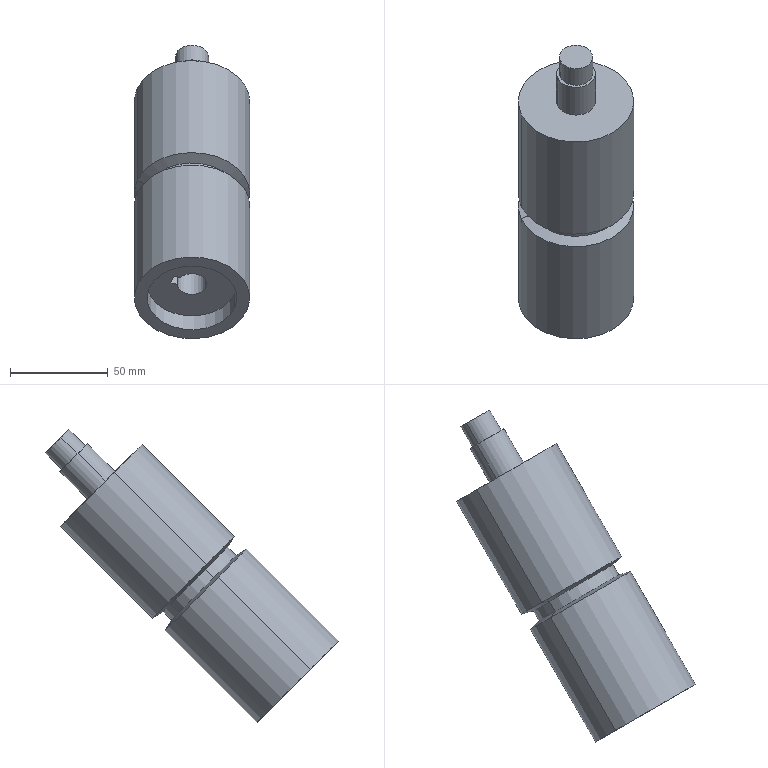Component | SolidWorks | AssemblyDriveAxis-1_DriveRoller-1 | 1 solid | 26 faces | box 59 x 149.91 x 149.91 mm | volume 368541 mm3 | cylinder 13 | plane 9 | cone 4 | commonest cylinder face diameters 59 x4 46 x2 47 x2 20 x2 17 x2 15 x1
build123d program:
from build123d import *

# Parameters (mm, degrees)
SKETCH2_W          = 5
SKETCH2_H          = 6.09
CUT_EXTRUDE1_DEPTH = 23.5


with BuildPart() as part:
    # Sketch1 → Revolve1 (revolve)
    with BuildSketch(Plane.XY, mode=Mode.PRIVATE) as revolve1_sk:
        Polygon((0, 0), (0, 8.5), (12, 8.5), (12, 10), (32, 10), (32, 29.5), (98.5, 29.5), (100, 23.5), (106, 23.5), (107.5, 29.5), (174, 29.5), (174, 23), (164, 23), (164, 7.5), (140.5, 7.5), (140.5, 0), align=None)
    revolve(revolve1_sk.sketch.rotate(Axis((0, 0, 0), (1, 0, 0)), 180), axis=Axis((0, 0, 0), (1, 0, 0)))

    # Sketch2 → Cut-Extrude1 (cut)
    with BuildSketch(Plane(origin=(164, 0, 0), x_dir=(0, 0, -1), z_dir=(1, 0, 0))):
        with Locations((0, -7.455)):
            Rectangle(SKETCH2_W, SKETCH2_H)
    extrude(amount=-CUT_EXTRUDE1_DEPTH, mode=Mode.SUBTRACT)


solid = part.part

# Placed as in the assembly
solid = solid.moved(Location((-102, 782.054, 414.962), (45, 18.175, -90)))
STEP:
#1=COLOUR_RGB('',0.7922,0.8196,0.9333);
#2=FILL_AREA_STYLE_COLOUR('',#1);
#3=FILL_AREA_STYLE('',(#2));
#4=SURFACE_STYLE_FILL_AREA(#3);
#5=SURFACE_SIDE_STYLE('',(#4));
#6=SURFACE_STYLE_USAGE(.BOTH.,#5);
#7=PRESENTATION_STYLE_ASSIGNMENT((#6));
#8=CARTESIAN_POINT('',(-3.155,26.145,11.293));
#9=VERTEX_POINT('',#8);
#10=CARTESIAN_POINT('',(-4.876,25.746,11.693));
#11=VERTEX_POINT('',#10);
#12=CARTESIAN_POINT('',(-4.016,25.946,11.493));
#13=DIRECTION('',(-0.,0.7071,0.7071));
#14=DIRECTION('',(-0.9501,-0.2206,0.2206));
#15=AXIS2_PLACEMENT_3D('',#12,#13,#14);
#16=CIRCLE('',#15,0.9055);
#17=EDGE_CURVE('',#9,#11,#16,.T.);
#18=ORIENTED_EDGE('',*,*,#17,.F.);
#19=CARTESIAN_POINT('',(-3.155,26.424,11.572));
#20=VERTEX_POINT('',#19);
#21=CARTESIAN_POINT('',(-3.155,30.989,16.137));
#22=DIRECTION('',(-0.,0.7071,0.7071));
#23=VECTOR('',#22,39.37);
#24=LINE('',#21,#23);
#25=EDGE_CURVE('',#9,#20,#24,.T.);
#26=ORIENTED_EDGE('',*,*,#25,.T.);
#27=CARTESIAN_POINT('',(-4.876,26.024,11.971));
#28=VERTEX_POINT('',#27);
#29=CARTESIAN_POINT('',(-4.016,26.224,11.772));
#30=DIRECTION('',(-0.,0.7071,0.7071));
#31=DIRECTION('',(-0.9501,-0.2206,0.2206));
#32=AXIS2_PLACEMENT_3D('',#29,#30,#31);
#33=CIRCLE('',#32,0.9055);
#34=EDGE_CURVE('',#20,#28,#33,.T.);
#35=ORIENTED_EDGE('',*,*,#34,.T.);
#36=CARTESIAN_POINT('',(-4.876,30.59,16.537));
#37=DIRECTION('',(-0.,0.7071,0.7071));
#38=VECTOR('',#37,39.37);
#39=LINE('',#36,#38);
#40=EDGE_CURVE('',#11,#28,#39,.T.);
#41=ORIENTED_EDGE('',*,*,#40,.F.);
#42=EDGE_LOOP('',(#18,#26,#35,#41));
#43=FACE_OUTER_BOUND('',#42,.T.);
#44=CARTESIAN_POINT('',(-4.016,30.79,16.337));
#45=DIRECTION('',(-0.,0.7071,0.7071));
#46=DIRECTION('',(-0.9501,-0.2206,0.2206));
#47=AXIS2_PLACEMENT_3D('',#44,#45,#46);
#48=CYLINDRICAL_SURFACE('',#47,0.9055);
#49=ADVANCED_FACE('',(#43),#48,.F.);
#50=CARTESIAN_POINT('',(-5.119,25.689,11.749));
#51=VERTEX_POINT('',#50);
#52=CARTESIAN_POINT('',(-2.912,26.202,11.237));
#53=VERTEX_POINT('',#52);
#54=CARTESIAN_POINT('',(-4.016,25.946,11.493));
#55=DIRECTION('',(-0.,0.7071,0.7071));
#56=DIRECTION('',(-0.9501,-0.2206,0.2206));
#57=AXIS2_PLACEMENT_3D('',#54,#55,#56);
#58=CIRCLE('',#57,1.161);
#59=EDGE_CURVE('',#51,#53,#58,.T.);
#60=ORIENTED_EDGE('',*,*,#59,.T.);
#61=CARTESIAN_POINT('',(-2.912,28.053,13.088));
#62=VERTEX_POINT('',#61);
#63=CARTESIAN_POINT('',(-2.912,31.046,16.081));
#64=DIRECTION('',(-0.,0.7071,0.7071));
#65=VECTOR('',#64,39.37);
#66=LINE('',#63,#65);
#67=EDGE_CURVE('',#53,#62,#66,.T.);
#68=ORIENTED_EDGE('',*,*,#67,.T.);
#69=CARTESIAN_POINT('',(-5.119,27.541,13.601));
#70=VERTEX_POINT('',#69);
#71=CARTESIAN_POINT('',(-4.016,27.797,13.344));
#72=DIRECTION('',(-0.,0.7071,0.7071));
#73=DIRECTION('',(-0.9501,-0.2206,0.2206));
#74=AXIS2_PLACEMENT_3D('',#71,#72,#73);
#75=CIRCLE('',#74,1.161);
#76=EDGE_CURVE('',#70,#62,#75,.T.);
#77=ORIENTED_EDGE('',*,*,#76,.F.);
#78=CARTESIAN_POINT('',(-5.119,30.533,16.593));
#79=DIRECTION('',(-0.,0.7071,0.7071));
#80=VECTOR('',#79,39.37);
#81=LINE('',#78,#80);
#82=EDGE_CURVE('',#51,#70,#81,.T.);
#83=ORIENTED_EDGE('',*,*,#82,.F.);
#84=EDGE_LOOP('',(#60,#68,#77,#83));
#85=FACE_OUTER_BOUND('',#84,.T.);
#86=CARTESIAN_POINT('',(-4.016,30.79,16.337));
#87=DIRECTION('',(-0.,0.7071,0.7071));
#88=DIRECTION('',(-0.9501,-0.2206,0.2206));
#89=AXIS2_PLACEMENT_3D('',#86,#87,#88);
#90=CYLINDRICAL_SURFACE('',#89,1.161);
#91=ADVANCED_FACE('',(#85),#90,.T.);
#92=CARTESIAN_POINT('',(-4.895,27.635,13.59));
#93=VERTEX_POINT('',#92);
#94=CARTESIAN_POINT('',(-3.137,28.043,13.182));
#95=VERTEX_POINT('',#94);
#96=CARTESIAN_POINT('',(-4.016,27.839,13.386));
#97=DIRECTION('',(-0.,0.7071,0.7071));
#98=DIRECTION('',(-0.9501,-0.2206,0.2206));
#99=AXIS2_PLACEMENT_3D('',#96,#97,#98);
#100=CIRCLE('',#99,0.9252);
#101=EDGE_CURVE('',#93,#95,#100,.T.);
#102=ORIENTED_EDGE('',*,*,#101,.F.);
#103=CARTESIAN_POINT('',(-5.119,27.541,13.601));
#104=DIRECTION('',(-0.9217,-0.3855,0.04248));
#105=VECTOR('',#104,39.37);
#106=LINE('',#103,#105);
#107=EDGE_CURVE('',#93,#70,#106,.T.);
#108=ORIENTED_EDGE('',*,*,#107,.T.);
#109=ORIENTED_EDGE('',*,*,#76,.T.);
#110=CARTESIAN_POINT('',(-2.912,28.053,13.088));
#111=DIRECTION('',(0.9217,0.04248,-0.3855));
#112=VECTOR('',#111,39.37);
#113=LINE('',#110,#112);
#114=EDGE_CURVE('',#95,#62,#113,.T.);
#115=ORIENTED_EDGE('',*,*,#114,.F.);
#116=EDGE_LOOP('',(#102,#108,#109,#115));
#117=FACE_OUTER_BOUND('',#116,.T.);
#118=CARTESIAN_POINT('',(-4.016,27.797,13.344));
#119=DIRECTION('',(0.,-0.7071,-0.7071));
#120=DIRECTION('',(0.9501,0.2206,-0.2206));
#121=AXIS2_PLACEMENT_3D('',#118,#119,#120);
#122=CONICAL_SURFACE('',#121,1.161,1.326);
#123=ADVANCED_FACE('',(#117),#122,.T.);
#124=ORIENTED_EDGE('',*,*,#101,.T.);
#125=CARTESIAN_POINT('',(-3.137,28.21,13.349));
#126=VERTEX_POINT('',#125);
#127=CARTESIAN_POINT('',(-3.137,30.994,16.133));
#128=DIRECTION('',(-0.,0.7071,0.7071));
#129=VECTOR('',#128,39.37);
#130=LINE('',#127,#129);
#131=EDGE_CURVE('',#95,#126,#130,.T.);
#132=ORIENTED_EDGE('',*,*,#131,.T.);
#133=CARTESIAN_POINT('',(-4.895,27.802,13.757));
#134=VERTEX_POINT('',#133);
#135=CARTESIAN_POINT('',(-4.016,28.006,13.553));
#136=DIRECTION('',(-0.,0.7071,0.7071));
#137=DIRECTION('',(-0.9501,-0.2206,0.2206));
#138=AXIS2_PLACEMENT_3D('',#135,#136,#137);
#139=CIRCLE('',#138,0.9252);
#140=EDGE_CURVE('',#134,#126,#139,.T.);
#141=ORIENTED_EDGE('',*,*,#140,.F.);
#142=CARTESIAN_POINT('',(-4.895,30.585,16.541));
#143=DIRECTION('',(-0.,0.7071,0.7071));
#144=VECTOR('',#143,39.37);
#145=LINE('',#142,#144);
#146=EDGE_CURVE('',#93,#134,#145,.T.);
#147=ORIENTED_EDGE('',*,*,#146,.F.);
#148=EDGE_LOOP('',(#124,#132,#141,#147));
#149=FACE_OUTER_BOUND('',#148,.T.);
#150=CARTESIAN_POINT('',(-4.016,30.79,16.337));
#151=DIRECTION('',(-0.,0.7071,0.7071));
#152=DIRECTION('',(-0.9501,-0.2206,0.2206));
#153=AXIS2_PLACEMENT_3D('',#150,#151,#152);
#154=CYLINDRICAL_SURFACE('',#153,0.9252);
#155=ADVANCED_FACE('',(#149),#154,.T.);
#156=ORIENTED_EDGE('',*,*,#140,.T.);
#157=CARTESIAN_POINT('',(-2.912,28.304,13.339));
#158=VERTEX_POINT('',#157);
#159=CARTESIAN_POINT('',(-3.137,28.21,13.349));
#160=DIRECTION('',(0.9217,0.3855,-0.04248));
#161=VECTOR('',#160,39.37);
#162=LINE('',#159,#161);
#163=EDGE_CURVE('',#126,#158,#162,.T.);
#164=ORIENTED_EDGE('',*,*,#163,.T.);
#165=CARTESIAN_POINT('',(-5.119,27.791,13.851));
#166=VERTEX_POINT('',#165);
#167=CARTESIAN_POINT('',(-4.016,28.047,13.595));
#168=DIRECTION('',(-0.,0.7071,0.7071));
#169=DIRECTION('',(-0.9501,-0.2206,0.2206));
#170=AXIS2_PLACEMENT_3D('',#167,#168,#169);
#171=CIRCLE('',#170,1.161);
#172=EDGE_CURVE('',#166,#158,#171,.T.);
#173=ORIENTED_EDGE('',*,*,#172,.F.);
#174=CARTESIAN_POINT('',(-4.895,27.802,13.757));
#175=DIRECTION('',(-0.9217,-0.04248,0.3855));
#176=VECTOR('',#175,39.37);
#177=LINE('',#174,#176);
#178=EDGE_CURVE('',#134,#166,#177,.T.);
#179=ORIENTED_EDGE('',*,*,#178,.F.);
#180=EDGE_LOOP('',(#156,#164,#173,#179));
#181=FACE_OUTER_BOUND('',#180,.T.);
#182=CARTESIAN_POINT('',(-4.016,28.006,13.553));
#183=DIRECTION('',(-0.,0.7071,0.7071));
#184=DIRECTION('',(-0.9501,-0.2206,0.2206));
#185=AXIS2_PLACEMENT_3D('',#182,#183,#184);
#186=CONICAL_SURFACE('',#185,0.9252,1.326);
#187=ADVANCED_FACE('',(#181),#186,.T.);
#188=ORIENTED_EDGE('',*,*,#172,.T.);
#189=CARTESIAN_POINT('',(-2.912,30.155,15.19));
#190=VERTEX_POINT('',#189);
#191=CARTESIAN_POINT('',(-2.912,31.046,16.081));
#192=DIRECTION('',(-0.,0.7071,0.7071));
#193=VECTOR('',#192,39.37);
#194=LINE('',#191,#193);
#195=EDGE_CURVE('',#158,#190,#194,.T.);
#196=ORIENTED_EDGE('',*,*,#195,.T.);
#197=CARTESIAN_POINT('',(-5.119,29.643,15.702));
#198=VERTEX_POINT('',#197);
#199=CARTESIAN_POINT('',(-4.016,29.899,15.446));
#200=DIRECTION('',(-0.,0.7071,0.7071));
#201=DIRECTION('',(-0.9501,-0.2206,0.2206));
#202=AXIS2_PLACEMENT_3D('',#199,#200,#201);
#203=CIRCLE('',#202,1.161);
#204=EDGE_CURVE('',#198,#190,#203,.T.);
#205=ORIENTED_EDGE('',*,*,#204,.F.);
#206=CARTESIAN_POINT('',(-5.119,30.533,16.593));
#207=DIRECTION('',(-0.,0.7071,0.7071));
#208=VECTOR('',#207,39.37);
#209=LINE('',#206,#208);
#210=EDGE_CURVE('',#166,#198,#209,.T.);
#211=ORIENTED_EDGE('',*,*,#210,.F.);
#212=EDGE_LOOP('',(#188,#196,#205,#211));
#213=FACE_OUTER_BOUND('',#212,.T.);
#214=CARTESIAN_POINT('',(-4.016,30.79,16.337));
#215=DIRECTION('',(-0.,0.7071,0.7071));
#216=DIRECTION('',(-0.9501,-0.2206,0.2206));
#217=AXIS2_PLACEMENT_3D('',#214,#215,#216);
#218=CYLINDRICAL_SURFACE('',#217,1.161);
#219=ADVANCED_FACE('',(#213),#218,.T.);
#220=CARTESIAN_POINT('',(-4.39,29.812,15.533));
#221=VERTEX_POINT('',#220);
#222=CARTESIAN_POINT('',(-3.642,29.986,15.359));
#223=VERTEX_POINT('',#222);
#224=CARTESIAN_POINT('',(-4.016,29.899,15.446));
#225=DIRECTION('',(-0.,0.7071,0.7071));
#226=DIRECTION('',(-0.9501,-0.2206,0.2206));
#227=AXIS2_PLACEMENT_3D('',#224,#225,#226);
#228=CIRCLE('',#227,0.3937);
#229=EDGE_CURVE('',#221,#223,#228,.T.);
#230=ORIENTED_EDGE('',*,*,#229,.T.);
#231=CARTESIAN_POINT('',(-3.642,30.542,15.916));
#232=VERTEX_POINT('',#231);
#233=CARTESIAN_POINT('',(-3.642,30.876,16.25));
#234=DIRECTION('',(-0.,0.7071,0.7071));
#235=VECTOR('',#234,39.37);
#236=LINE('',#233,#235);
#237=EDGE_CURVE('',#223,#232,#236,.T.);
#238=ORIENTED_EDGE('',*,*,#237,.T.);
#239=CARTESIAN_POINT('',(-4.39,30.369,16.09));
#240=VERTEX_POINT('',#239);
#241=CARTESIAN_POINT('',(-4.016,30.455,16.003));
#242=DIRECTION('',(-0.,0.7071,0.7071));
#243=DIRECTION('',(-0.9501,-0.2206,0.2206));
#244=AXIS2_PLACEMENT_3D('',#241,#242,#243);
#245=CIRCLE('',#244,0.3937);
#246=EDGE_CURVE('',#240,#232,#245,.T.);
#247=ORIENTED_EDGE('',*,*,#246,.F.);
#248=CARTESIAN_POINT('',(-4.39,30.703,16.424));
#249=DIRECTION('',(-0.,0.7071,0.7071));
#250=VECTOR('',#249,39.37);
#251=LINE('',#248,#250);
#252=EDGE_CURVE('',#221,#240,#251,.T.);
#253=ORIENTED_EDGE('',*,*,#252,.F.);
#254=EDGE_LOOP('',(#230,#238,#247,#253));
#255=FACE_OUTER_BOUND('',#254,.T.);
#256=CARTESIAN_POINT('',(-4.016,30.79,16.337));
#257=DIRECTION('',(-0.,0.7071,0.7071));
#258=DIRECTION('',(-0.9501,-0.2206,0.2206));
#259=AXIS2_PLACEMENT_3D('',#256,#257,#258);
#260=CYLINDRICAL_SURFACE('',#259,0.3937);
#261=ADVANCED_FACE('',(#255),#260,.T.);
#262=CARTESIAN_POINT('',(-4.334,30.382,16.077));
#263=VERTEX_POINT('',#262);
#264=CARTESIAN_POINT('',(-3.698,30.529,15.929));
#265=VERTEX_POINT('',#264);
#266=CARTESIAN_POINT('',(-4.016,30.455,16.003));
#267=DIRECTION('',(-0.,0.7071,0.7071));
#268=DIRECTION('',(-0.9501,-0.2206,0.2206));
#269=AXIS2_PLACEMENT_3D('',#266,#267,#268);
#270=CIRCLE('',#269,0.3346);
#271=EDGE_CURVE('',#263,#265,#270,.T.);
#272=ORIENTED_EDGE('',*,*,#271,.T.);
#273=CARTESIAN_POINT('',(-3.698,30.863,16.263));
#274=VERTEX_POINT('',#273);
#275=CARTESIAN_POINT('',(-3.698,30.863,16.263));
#276=DIRECTION('',(-0.,0.7071,0.7071));
#277=VECTOR('',#276,39.37);
#278=LINE('',#275,#277);
#279=EDGE_CURVE('',#265,#274,#278,.T.);
#280=ORIENTED_EDGE('',*,*,#279,.T.);
#281=CARTESIAN_POINT('',(-4.334,30.716,16.411));
#282=VERTEX_POINT('',#281);
#283=CARTESIAN_POINT('',(-4.016,30.79,16.337));
#284=DIRECTION('',(-0.,0.7071,0.7071));
#285=DIRECTION('',(-0.9501,-0.2206,0.2206));
#286=AXIS2_PLACEMENT_3D('',#283,#284,#285);
#287=CIRCLE('',#286,0.3346);
#288=EDGE_CURVE('',#282,#274,#287,.T.);
#289=ORIENTED_EDGE('',*,*,#288,.F.);
#290=CARTESIAN_POINT('',(-4.334,30.716,16.411));
#291=DIRECTION('',(-0.,0.7071,0.7071));
#292=VECTOR('',#291,39.37);
#293=LINE('',#290,#292);
#294=EDGE_CURVE('',#263,#282,#293,.T.);
#295=ORIENTED_EDGE('',*,*,#294,.F.);
#296=EDGE_LOOP('',(#272,#280,#289,#295));
#297=FACE_OUTER_BOUND('',#296,.T.);
#298=CARTESIAN_POINT('',(-4.016,30.79,16.337));
#299=DIRECTION('',(-0.,0.7071,0.7071));
#300=DIRECTION('',(-0.9501,-0.2206,0.2206));
#301=AXIS2_PLACEMENT_3D('',#298,#299,#300);
#302=CYLINDRICAL_SURFACE('',#301,0.3346);
#303=ADVANCED_FACE('',(#297),#302,.T.);
#304=ORIENTED_EDGE('',*,*,#288,.T.);
#305=CARTESIAN_POINT('',(-4.016,30.79,16.337));
#306=DIRECTION('',(-0.,0.7071,0.7071));
#307=DIRECTION('',(-0.9501,-0.2206,0.2206));
#308=AXIS2_PLACEMENT_3D('',#305,#306,#307);
#309=CIRCLE('',#308,0.3346);
#310=EDGE_CURVE('',#274,#282,#309,.T.);
#311=ORIENTED_EDGE('',*,*,#310,.T.);
#312=EDGE_LOOP('',(#304,#311));
#313=FACE_OUTER_BOUND('',#312,.T.);
#314=CARTESIAN_POINT('',(-4.016,30.79,16.337));
#315=DIRECTION('',(0.,-0.7071,-0.7071));
#316=DIRECTION('',(0.9501,0.2206,-0.2206));
#317=AXIS2_PLACEMENT_3D('',#314,#315,#316);
#318=PLANE('',#317);
#319=ADVANCED_FACE('',(#313),#318,.F.);
#320=ORIENTED_EDGE('',*,*,#279,.F.);
#321=CARTESIAN_POINT('',(-4.016,30.455,16.003));
#322=DIRECTION('',(-0.,0.7071,0.7071));
#323=DIRECTION('',(-0.9501,-0.2206,0.2206));
#324=AXIS2_PLACEMENT_3D('',#321,#322,#323);
#325=CIRCLE('',#324,0.3346);
#326=EDGE_CURVE('',#265,#263,#325,.T.);
#327=ORIENTED_EDGE('',*,*,#326,.T.);
#328=ORIENTED_EDGE('',*,*,#294,.T.);
#329=ORIENTED_EDGE('',*,*,#310,.F.);
#330=EDGE_LOOP('',(#320,#327,#328,#329));
#331=FACE_OUTER_BOUND('',#330,.T.);
#332=CARTESIAN_POINT('',(-4.016,30.79,16.337));
#333=DIRECTION('',(-0.,0.7071,0.7071));
#334=DIRECTION('',(-0.9501,-0.2206,0.2206));
#335=AXIS2_PLACEMENT_3D('',#332,#333,#334);
#336=CYLINDRICAL_SURFACE('',#335,0.3346);
#337=ADVANCED_FACE('',(#331),#336,.T.);
#338=ORIENTED_EDGE('',*,*,#271,.F.);
#339=ORIENTED_EDGE('',*,*,#326,.F.);
#340=EDGE_LOOP('',(#338,#339));
#341=FACE_BOUND('',#340,.T.);
#342=ORIENTED_EDGE('',*,*,#246,.T.);
#343=CARTESIAN_POINT('',(-4.016,30.455,16.003));
#344=DIRECTION('',(-0.,0.7071,0.7071));
#345=DIRECTION('',(-0.9501,-0.2206,0.2206));
#346=AXIS2_PLACEMENT_3D('',#343,#344,#345);
#347=CIRCLE('',#346,0.3937);
#348=EDGE_CURVE('',#232,#240,#347,.T.);
#349=ORIENTED_EDGE('',*,*,#348,.T.);
#350=EDGE_LOOP('',(#342,#349));
#351=FACE_OUTER_BOUND('',#350,.T.);
#352=CARTESIAN_POINT('',(-3.698,30.529,15.929));
#353=DIRECTION('',(0.,-0.7071,-0.7071));
#354=DIRECTION('',(0.9501,0.2206,-0.2206));
#355=AXIS2_PLACEMENT_3D('',#352,#353,#354);
#356=PLANE('',#355);
#357=ADVANCED_FACE('',(#341,#351),#356,.F.);
#358=ORIENTED_EDGE('',*,*,#237,.F.);
#359=CARTESIAN_POINT('',(-4.016,29.899,15.446));
#360=DIRECTION('',(-0.,0.7071,0.7071));
#361=DIRECTION('',(-0.9501,-0.2206,0.2206));
#362=AXIS2_PLACEMENT_3D('',#359,#360,#361);
#363=CIRCLE('',#362,0.3937);
#364=EDGE_CURVE('',#223,#221,#363,.T.);
#365=ORIENTED_EDGE('',*,*,#364,.T.);
#366=ORIENTED_EDGE('',*,*,#252,.T.);
#367=ORIENTED_EDGE('',*,*,#348,.F.);
#368=EDGE_LOOP('',(#358,#365,#366,#367));
#369=FACE_OUTER_BOUND('',#368,.T.);
#370=CARTESIAN_POINT('',(-4.016,30.79,16.337));
#371=DIRECTION('',(-0.,0.7071,0.7071));
#372=DIRECTION('',(-0.9501,-0.2206,0.2206));
#373=AXIS2_PLACEMENT_3D('',#370,#371,#372);
#374=CYLINDRICAL_SURFACE('',#373,0.3937);
#375=ADVANCED_FACE('',(#369),#374,.T.);
#376=ORIENTED_EDGE('',*,*,#229,.F.);
#377=ORIENTED_EDGE('',*,*,#364,.F.);
#378=EDGE_LOOP('',(#376,#377));
#379=FACE_BOUND('',#378,.T.);
#380=ORIENTED_EDGE('',*,*,#204,.T.);
#381=CARTESIAN_POINT('',(-4.016,29.899,15.446));
#382=DIRECTION('',(-0.,0.7071,0.7071));
#383=DIRECTION('',(-0.9501,-0.2206,0.2206));
#384=AXIS2_PLACEMENT_3D('',#381,#382,#383);
#385=CIRCLE('',#384,1.161);
#386=EDGE_CURVE('',#190,#198,#385,.T.);
#387=ORIENTED_EDGE('',*,*,#386,.T.);
#388=EDGE_LOOP('',(#380,#387));
#389=FACE_OUTER_BOUND('',#388,.T.);
#390=CARTESIAN_POINT('',(-3.642,29.986,15.359));
#391=DIRECTION('',(0.,-0.7071,-0.7071));
#392=DIRECTION('',(0.9501,0.2206,-0.2206));
#393=AXIS2_PLACEMENT_3D('',#390,#391,#392);
#394=PLANE('',#393);
#395=ADVANCED_FACE('',(#379,#389),#394,.F.);
#396=ORIENTED_EDGE('',*,*,#195,.F.);
#397=CARTESIAN_POINT('',(-4.016,28.047,13.595));
#398=DIRECTION('',(-0.,0.7071,0.7071));
#399=DIRECTION('',(-0.9501,-0.2206,0.2206));
#400=AXIS2_PLACEMENT_3D('',#397,#398,#399);
#401=CIRCLE('',#400,1.161);
#402=EDGE_CURVE('',#158,#166,#401,.T.);
#403=ORIENTED_EDGE('',*,*,#402,.T.);
#404=ORIENTED_EDGE('',*,*,#210,.T.);
#405=ORIENTED_EDGE('',*,*,#386,.F.);
#406=EDGE_LOOP('',(#396,#403,#404,#405));
#407=FACE_OUTER_BOUND('',#406,.T.);
#408=CARTESIAN_POINT('',(-4.016,30.79,16.337));
#409=DIRECTION('',(-0.,0.7071,0.7071));
#410=DIRECTION('',(-0.9501,-0.2206,0.2206));
#411=AXIS2_PLACEMENT_3D('',#408,#409,#410);
#412=CYLINDRICAL_SURFACE('',#411,1.161);
#413=ADVANCED_FACE('',(#407),#412,.T.);
#414=ORIENTED_EDGE('',*,*,#163,.F.);
#415=CARTESIAN_POINT('',(-4.016,28.006,13.553));
#416=DIRECTION('',(-0.,0.7071,0.7071));
#417=DIRECTION('',(-0.9501,-0.2206,0.2206));
#418=AXIS2_PLACEMENT_3D('',#415,#416,#417);
#419=CIRCLE('',#418,0.9252);
#420=EDGE_CURVE('',#126,#134,#419,.T.);
#421=ORIENTED_EDGE('',*,*,#420,.T.);
#422=ORIENTED_EDGE('',*,*,#178,.T.);
#423=ORIENTED_EDGE('',*,*,#402,.F.);
#424=EDGE_LOOP('',(#414,#421,#422,#423));
#425=FACE_OUTER_BOUND('',#424,.T.);
#426=CARTESIAN_POINT('',(-4.016,28.006,13.553));
#427=DIRECTION('',(-0.,0.7071,0.7071));
#428=DIRECTION('',(-0.9501,-0.2206,0.2206));
#429=AXIS2_PLACEMENT_3D('',#426,#427,#428);
#430=CONICAL_SURFACE('',#429,0.9252,1.326);
#431=ADVANCED_FACE('',(#425),#430,.T.);
#432=ORIENTED_EDGE('',*,*,#131,.F.);
#433=CARTESIAN_POINT('',(-4.016,27.839,13.386));
#434=DIRECTION('',(-0.,0.7071,0.7071));
#435=DIRECTION('',(-0.9501,-0.2206,0.2206));
#436=AXIS2_PLACEMENT_3D('',#433,#434,#435);
#437=CIRCLE('',#436,0.9252);
#438=EDGE_CURVE('',#95,#93,#437,.T.);
#439=ORIENTED_EDGE('',*,*,#438,.T.);
#440=ORIENTED_EDGE('',*,*,#146,.T.);
#441=ORIENTED_EDGE('',*,*,#420,.F.);
#442=EDGE_LOOP('',(#432,#439,#440,#441));
#443=FACE_OUTER_BOUND('',#442,.T.);
#444=CARTESIAN_POINT('',(-4.016,30.79,16.337));
#445=DIRECTION('',(-0.,0.7071,0.7071));
#446=DIRECTION('',(-0.9501,-0.2206,0.2206));
#447=AXIS2_PLACEMENT_3D('',#444,#445,#446);
#448=CYLINDRICAL_SURFACE('',#447,0.9252);
#449=ADVANCED_FACE('',(#443),#448,.T.);
#450=ORIENTED_EDGE('',*,*,#107,.F.);
#451=ORIENTED_EDGE('',*,*,#438,.F.);
#452=ORIENTED_EDGE('',*,*,#114,.T.);
#453=CARTESIAN_POINT('',(-4.016,27.797,13.344));
#454=DIRECTION('',(-0.,0.7071,0.7071));
#455=DIRECTION('',(-0.9501,-0.2206,0.2206));
#456=AXIS2_PLACEMENT_3D('',#453,#454,#455);
#457=CIRCLE('',#456,1.161);
#458=EDGE_CURVE('',#62,#70,#457,.T.);
#459=ORIENTED_EDGE('',*,*,#458,.T.);
#460=EDGE_LOOP('',(#450,#451,#452,#459));
#461=FACE_OUTER_BOUND('',#460,.T.);
#462=CARTESIAN_POINT('',(-4.016,27.797,13.344));
#463=DIRECTION('',(0.,-0.7071,-0.7071));
#464=DIRECTION('',(0.9501,0.2206,-0.2206));
#465=AXIS2_PLACEMENT_3D('',#462,#463,#464);
#466=CONICAL_SURFACE('',#465,1.161,1.326);
#467=ADVANCED_FACE('',(#461),#466,.T.);
#468=ORIENTED_EDGE('',*,*,#67,.F.);
#469=CARTESIAN_POINT('',(-4.016,25.946,11.493));
#470=DIRECTION('',(-0.,0.7071,0.7071));
#471=DIRECTION('',(-0.9501,-0.2206,0.2206));
#472=AXIS2_PLACEMENT_3D('',#469,#470,#471);
#473=CIRCLE('',#472,1.161);
#474=EDGE_CURVE('',#53,#51,#473,.T.);
#475=ORIENTED_EDGE('',*,*,#474,.T.);
#476=ORIENTED_EDGE('',*,*,#82,.T.);
#477=ORIENTED_EDGE('',*,*,#458,.F.);
#478=EDGE_LOOP('',(#468,#475,#476,#477));
#479=FACE_OUTER_BOUND('',#478,.T.);
#480=CARTESIAN_POINT('',(-4.016,30.79,16.337));
#481=DIRECTION('',(-0.,0.7071,0.7071));
#482=DIRECTION('',(-0.9501,-0.2206,0.2206));
#483=AXIS2_PLACEMENT_3D('',#480,#481,#482);
#484=CYLINDRICAL_SURFACE('',#483,1.161);
#485=ADVANCED_FACE('',(#479),#484,.T.);
#486=ORIENTED_EDGE('',*,*,#59,.F.);
#487=ORIENTED_EDGE('',*,*,#474,.F.);
#488=EDGE_LOOP('',(#486,#487));
#489=FACE_OUTER_BOUND('',#488,.T.);
#490=CARTESIAN_POINT('',(-4.016,25.946,11.493));
#491=DIRECTION('',(-0.,0.7071,0.7071));
#492=DIRECTION('',(-0.9501,-0.2206,0.2206));
#493=AXIS2_PLACEMENT_3D('',#490,#491,#492);
#494=CIRCLE('',#493,0.9055);
#495=EDGE_CURVE('',#11,#9,#494,.T.);
#496=ORIENTED_EDGE('',*,*,#495,.T.);
#497=ORIENTED_EDGE('',*,*,#17,.T.);
#498=EDGE_LOOP('',(#496,#497));
#499=FACE_BOUND('',#498,.T.);
#500=CARTESIAN_POINT('',(-2.912,26.202,11.237));
#501=DIRECTION('',(-0.,0.7071,0.7071));
#502=DIRECTION('',(-0.9501,-0.2206,0.2206));
#503=AXIS2_PLACEMENT_3D('',#500,#501,#502);
#504=PLANE('',#503);
#505=ADVANCED_FACE('',(#489,#499),#504,.F.);
#506=ORIENTED_EDGE('',*,*,#25,.F.);
#507=ORIENTED_EDGE('',*,*,#495,.F.);
#508=ORIENTED_EDGE('',*,*,#40,.T.);
#509=CARTESIAN_POINT('',(-4.016,26.224,11.772));
#510=DIRECTION('',(-0.,0.7071,0.7071));
#511=DIRECTION('',(-0.9501,-0.2206,0.2206));
#512=AXIS2_PLACEMENT_3D('',#509,#510,#511);
#513=CIRCLE('',#512,0.9055);
#514=EDGE_CURVE('',#28,#20,#513,.T.);
#515=ORIENTED_EDGE('',*,*,#514,.T.);
#516=EDGE_LOOP('',(#506,#507,#508,#515));
#517=FACE_OUTER_BOUND('',#516,.T.);
#518=CARTESIAN_POINT('',(-4.016,30.79,16.337));
#519=DIRECTION('',(-0.,0.7071,0.7071));
#520=DIRECTION('',(-0.9501,-0.2206,0.2206));
#521=AXIS2_PLACEMENT_3D('',#518,#519,#520);
#522=CYLINDRICAL_SURFACE('',#521,0.9055);
#523=ADVANCED_FACE('',(#517),#522,.F.);
#524=ORIENTED_EDGE('',*,*,#514,.F.);
#525=ORIENTED_EDGE('',*,*,#34,.F.);
#526=EDGE_LOOP('',(#524,#525));
#527=FACE_OUTER_BOUND('',#526,.T.);
#528=CARTESIAN_POINT('',(-4.378,26.067,11.929));
#529=VERTEX_POINT('',#528);
#530=CARTESIAN_POINT('',(-4.439,26.199,11.797));
#531=VERTEX_POINT('',#530);
#532=CARTESIAN_POINT('',(-4.378,26.067,11.929));
#533=DIRECTION('',(-0.3119,0.6718,-0.6718));
#534=VECTOR('',#533,39.37);
#535=LINE('',#532,#534);
#536=EDGE_CURVE('',#529,#531,#535,.T.);
#537=ORIENTED_EDGE('',*,*,#536,.F.);
#538=CARTESIAN_POINT('',(-4.25,26.096,11.899));
#539=VERTEX_POINT('',#538);
#540=CARTESIAN_POINT('',(-4.15,26.12,11.876));
#541=DIRECTION('',(-0.9501,-0.2206,0.2206));
#542=VECTOR('',#541,39.37);
#543=LINE('',#540,#542);
#544=EDGE_CURVE('',#539,#529,#543,.T.);
#545=ORIENTED_EDGE('',*,*,#544,.F.);
#546=CARTESIAN_POINT('',(-4.311,26.229,11.767));
#547=VERTEX_POINT('',#546);
#548=CARTESIAN_POINT('',(-4.016,26.224,11.772));
#549=DIRECTION('',(-0.,0.7071,0.7071));
#550=DIRECTION('',(-0.9501,-0.2206,0.2206));
#551=AXIS2_PLACEMENT_3D('',#548,#549,#550);
#552=CIRCLE('',#551,0.2953);
#553=EDGE_CURVE('',#539,#547,#552,.T.);
#554=ORIENTED_EDGE('',*,*,#553,.T.);
#555=CARTESIAN_POINT('',(-4.439,26.199,11.797));
#556=DIRECTION('',(0.9501,0.2206,-0.2206));
#557=VECTOR('',#556,39.37);
#558=LINE('',#555,#557);
#559=EDGE_CURVE('',#531,#547,#558,.T.);
#560=ORIENTED_EDGE('',*,*,#559,.F.);
#561=EDGE_LOOP('',(#537,#545,#554,#560));
#562=FACE_BOUND('',#561,.T.);
#563=CARTESIAN_POINT('',(-3.155,26.424,11.572));
#564=DIRECTION('',(-0.,0.7071,0.7071));
#565=DIRECTION('',(-0.9501,-0.2206,0.2206));
#566=AXIS2_PLACEMENT_3D('',#563,#564,#565);
#567=PLANE('',#566);
#568=ADVANCED_FACE('',(#527,#562),#567,.F.);
#569=ORIENTED_EDGE('',*,*,#553,.F.);
#570=CARTESIAN_POINT('',(-4.25,26.751,12.553));
#571=VERTEX_POINT('',#570);
#572=CARTESIAN_POINT('',(-4.25,30.662,16.465));
#573=DIRECTION('',(-0.,0.7071,0.7071));
#574=VECTOR('',#573,39.37);
#575=LINE('',#572,#574);
#576=EDGE_CURVE('',#539,#571,#575,.T.);
#577=ORIENTED_EDGE('',*,*,#576,.T.);
#578=CARTESIAN_POINT('',(-4.311,26.883,12.421));
#579=VERTEX_POINT('',#578);
#580=CARTESIAN_POINT('',(-4.016,26.878,12.426));
#581=DIRECTION('',(-0.,0.7071,0.7071));
#582=DIRECTION('',(-0.9501,-0.2206,0.2206));
#583=AXIS2_PLACEMENT_3D('',#580,#581,#582);
#584=CIRCLE('',#583,0.2953);
#585=EDGE_CURVE('',#571,#579,#584,.T.);
#586=ORIENTED_EDGE('',*,*,#585,.T.);
#587=CARTESIAN_POINT('',(-4.311,30.794,16.332));
#588=DIRECTION('',(0.,-0.7071,-0.7071));
#589=VECTOR('',#588,39.37);
#590=LINE('',#587,#589);
#591=EDGE_CURVE('',#579,#547,#590,.T.);
#592=ORIENTED_EDGE('',*,*,#591,.T.);
#593=EDGE_LOOP('',(#569,#577,#586,#592));
#594=FACE_OUTER_BOUND('',#593,.T.);
#595=CARTESIAN_POINT('',(-4.016,30.79,16.337));
#596=DIRECTION('',(-0.,0.7071,0.7071));
#597=DIRECTION('',(-0.9501,-0.2206,0.2206));
#598=AXIS2_PLACEMENT_3D('',#595,#596,#597);
#599=CYLINDRICAL_SURFACE('',#598,0.2953);
#600=ADVANCED_FACE('',(#594),#599,.F.);
#601=ORIENTED_EDGE('',*,*,#585,.F.);
#602=CARTESIAN_POINT('',(-4.378,26.721,12.583));
#603=VERTEX_POINT('',#602);
#604=CARTESIAN_POINT('',(-4.15,26.774,12.53));
#605=DIRECTION('',(-0.9501,-0.2206,0.2206));
#606=VECTOR('',#605,39.37);
#607=LINE('',#604,#606);
#608=EDGE_CURVE('',#571,#603,#607,.T.);
#609=ORIENTED_EDGE('',*,*,#608,.T.);
#610=CARTESIAN_POINT('',(-4.439,26.853,12.451));
#611=VERTEX_POINT('',#610);
#612=CARTESIAN_POINT('',(-4.378,26.721,12.583));
#613=DIRECTION('',(-0.3119,0.6718,-0.6718));
#614=VECTOR('',#613,39.37);
#615=LINE('',#612,#614);
#616=EDGE_CURVE('',#603,#611,#615,.T.);
#617=ORIENTED_EDGE('',*,*,#616,.T.);
#618=CARTESIAN_POINT('',(-4.439,26.853,12.451));
#619=DIRECTION('',(0.9501,0.2206,-0.2206));
#620=VECTOR('',#619,39.37);
#621=LINE('',#618,#620);
#622=EDGE_CURVE('',#611,#579,#621,.T.);
#623=ORIENTED_EDGE('',*,*,#622,.T.);
#624=EDGE_LOOP('',(#601,#609,#617,#623));
#625=FACE_OUTER_BOUND('',#624,.T.);
#626=CARTESIAN_POINT('',(-3.735,26.943,12.361));
#627=DIRECTION('',(-0.,0.7071,0.7071));
#628=DIRECTION('',(-0.9501,-0.2206,0.2206));
#629=AXIS2_PLACEMENT_3D('',#626,#627,#628);
#630=PLANE('',#629);
#631=ADVANCED_FACE('',(#625),#630,.F.);
#632=ORIENTED_EDGE('',*,*,#544,.T.);
#633=CARTESIAN_POINT('',(-4.378,26.94,12.802));
#634=DIRECTION('',(0.,-0.7071,-0.7071));
#635=VECTOR('',#634,39.37);
#636=LINE('',#633,#635);
#637=EDGE_CURVE('',#603,#529,#636,.T.);
#638=ORIENTED_EDGE('',*,*,#637,.F.);
#639=ORIENTED_EDGE('',*,*,#608,.F.);
#640=ORIENTED_EDGE('',*,*,#576,.F.);
#641=EDGE_LOOP('',(#632,#638,#639,#640));
#642=FACE_OUTER_BOUND('',#641,.T.);
#643=CARTESIAN_POINT('',(-4.15,26.993,12.75));
#644=DIRECTION('',(0.3119,-0.6718,0.6718));
#645=DIRECTION('',(-0.9501,-0.2206,0.2206));
#646=AXIS2_PLACEMENT_3D('',#643,#644,#645);
#647=PLANE('',#646);
#648=ADVANCED_FACE('',(#642),#647,.F.);
#649=ORIENTED_EDGE('',*,*,#622,.F.);
#650=CARTESIAN_POINT('',(-4.439,27.072,12.67));
#651=DIRECTION('',(0.,-0.7071,-0.7071));
#652=VECTOR('',#651,39.37);
#653=LINE('',#650,#652);
#654=EDGE_CURVE('',#611,#531,#653,.T.);
#655=ORIENTED_EDGE('',*,*,#654,.T.);
#656=ORIENTED_EDGE('',*,*,#559,.T.);
#657=ORIENTED_EDGE('',*,*,#591,.F.);
#658=EDGE_LOOP('',(#649,#655,#656,#657));
#659=FACE_OUTER_BOUND('',#658,.T.);
#660=CARTESIAN_POINT('',(-4.439,27.072,12.67));
#661=DIRECTION('',(-0.3119,0.6718,-0.6718));
#662=DIRECTION('',(0.9501,0.2206,-0.2206));
#663=AXIS2_PLACEMENT_3D('',#660,#661,#662);
#664=PLANE('',#663);
#665=ADVANCED_FACE('',(#659),#664,.F.);
#666=ORIENTED_EDGE('',*,*,#637,.T.);
#667=ORIENTED_EDGE('',*,*,#536,.T.);
#668=ORIENTED_EDGE('',*,*,#654,.F.);
#669=ORIENTED_EDGE('',*,*,#616,.F.);
#670=EDGE_LOOP('',(#666,#667,#668,#669));
#671=FACE_OUTER_BOUND('',#670,.T.);
#672=CARTESIAN_POINT('',(-4.378,26.94,12.802));
#673=DIRECTION('',(-0.9501,-0.2206,0.2206));
#674=DIRECTION('',(-0.3119,0.6718,-0.6718));
#675=AXIS2_PLACEMENT_3D('',#672,#673,#674);
#676=PLANE('',#675);
#677=ADVANCED_FACE('',(#671),#676,.F.);
#678=CLOSED_SHELL('',(#49,#91,#123,#155,#187,#219,#261,#303,#319,#337,#357,#375,#395,#413,#431,#449,#467,#485,#505,#523,#568,#600,#631,#648,#665,#677));
#679=MANIFOLD_SOLID_BREP('',#678);
#680=STYLED_ITEM('',(#7),#679);
#681=PRESENTATION_LAYER_ASSIGNMENT('','',(#680));
#682=CARTESIAN_POINT('',(0.,0.,0.));
#683=DIRECTION('',(0.,0.,1.));
#684=DIRECTION('',(1.,0.,0.));
#685=AXIS2_PLACEMENT_3D('',#682,#683,#684);
#686=(LENGTH_UNIT()NAMED_UNIT(*)SI_UNIT($,.METRE.));
#687=LENGTH_MEASURE_WITH_UNIT(LENGTH_MEASURE(0.0254),#686);
#688=DIMENSIONAL_EXPONENTS(1.,0.,0.,0.,0.,0.,0.);
#689=(CONVERSION_BASED_UNIT('',#687)LENGTH_UNIT()NAMED_UNIT(#688));
#690=UNCERTAINTY_MEASURE_WITH_UNIT(LENGTH_MEASURE(0.00001),#689,'','');
#691=(NAMED_UNIT(*)PLANE_ANGLE_UNIT()SI_UNIT($,.RADIAN.));
#692=(NAMED_UNIT(*)SI_UNIT($,.STERADIAN.)SOLID_ANGLE_UNIT());
#693=(GEOMETRIC_REPRESENTATION_CONTEXT(3)GLOBAL_UNCERTAINTY_ASSIGNED_CONTEXT((#690))GLOBAL_UNIT_ASSIGNED_CONTEXT((#689,#691,#692))REPRESENTATION_CONTEXT('',''));
#694=ADVANCED_BREP_SHAPE_REPRESENTATION('',(#679,#685),#693);
#695=(LENGTH_UNIT()NAMED_UNIT(*)SI_UNIT($,.METRE.));
#696=LENGTH_MEASURE_WITH_UNIT(LENGTH_MEASURE(0.0254),#695);
#697=DIMENSIONAL_EXPONENTS(1.,0.,0.,0.,0.,0.,0.);
#698=(CONVERSION_BASED_UNIT('',#696)LENGTH_UNIT()NAMED_UNIT(#697));
#699=UNCERTAINTY_MEASURE_WITH_UNIT(LENGTH_MEASURE(0.00001),#698,'','');
#700=(NAMED_UNIT(*)PLANE_ANGLE_UNIT()SI_UNIT($,.RADIAN.));
#701=(NAMED_UNIT(*)SI_UNIT($,.STERADIAN.)SOLID_ANGLE_UNIT());
#702=(GEOMETRIC_REPRESENTATION_CONTEXT(3)GLOBAL_UNCERTAINTY_ASSIGNED_CONTEXT((#699))GLOBAL_UNIT_ASSIGNED_CONTEXT((#698,#700,#701))REPRESENTATION_CONTEXT('',''));
#703=MECHANICAL_DESIGN_GEOMETRIC_PRESENTATION_REPRESENTATION('',(#680),#702);